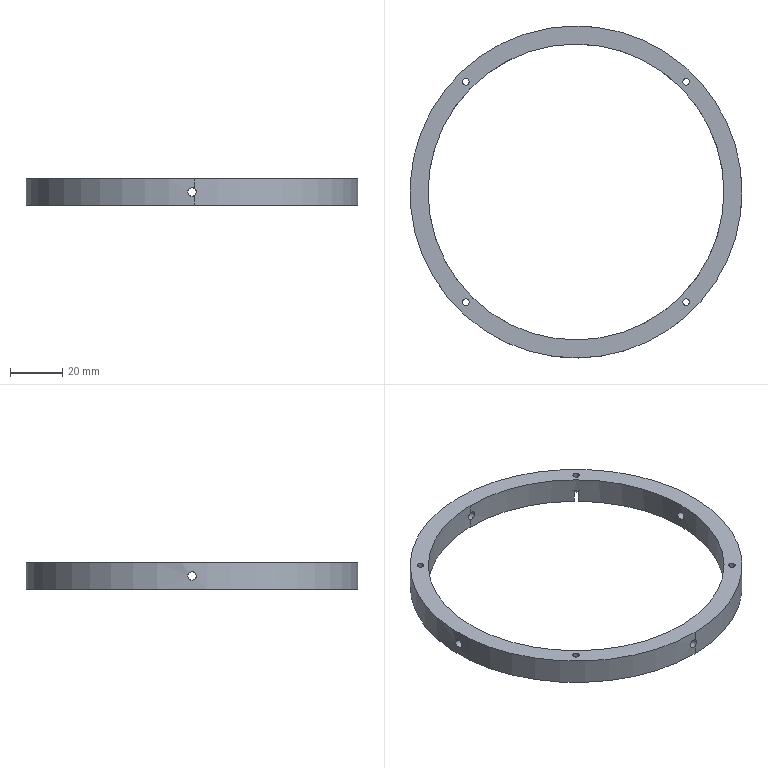CAM job | Mastercam | mm | 6 operations | part box 126.8 x 126.8 x 10
1. Contour (Ramp) | 4 - 4 平铣刀
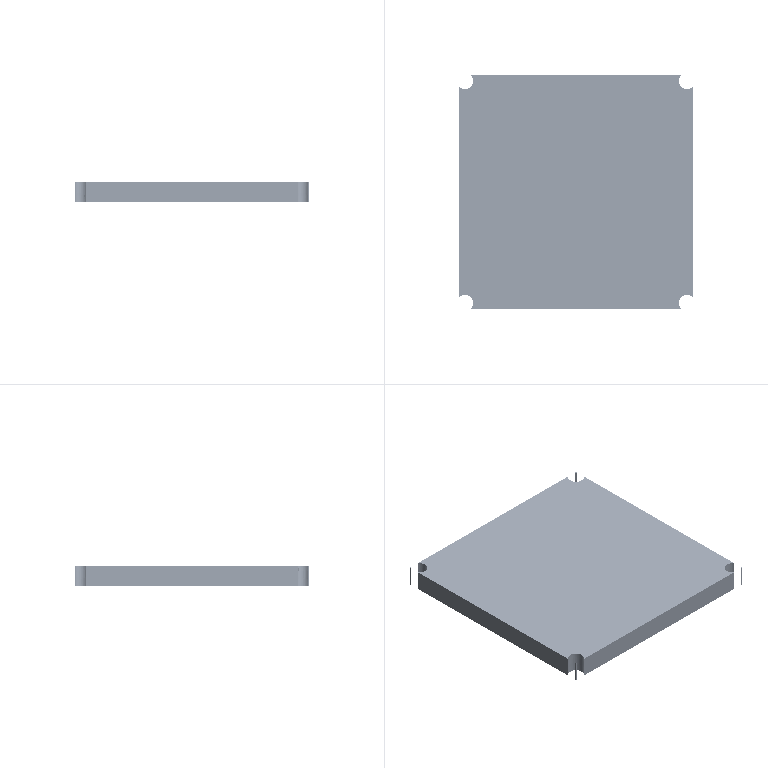2. Contour (2D) | 4 - 4 平铣刀
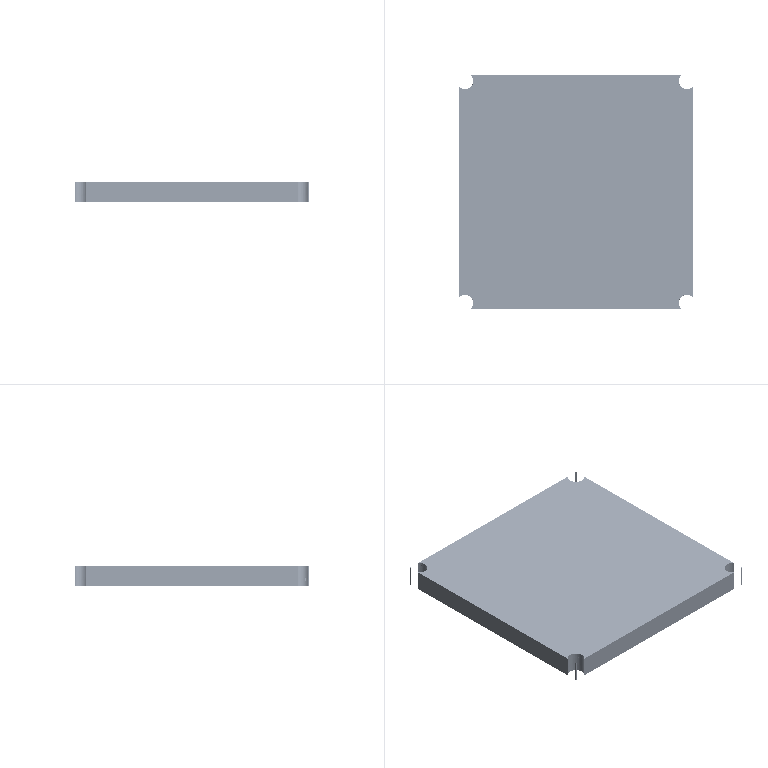3. Contour (2D chamfer) | 7 - 4 倒角刀
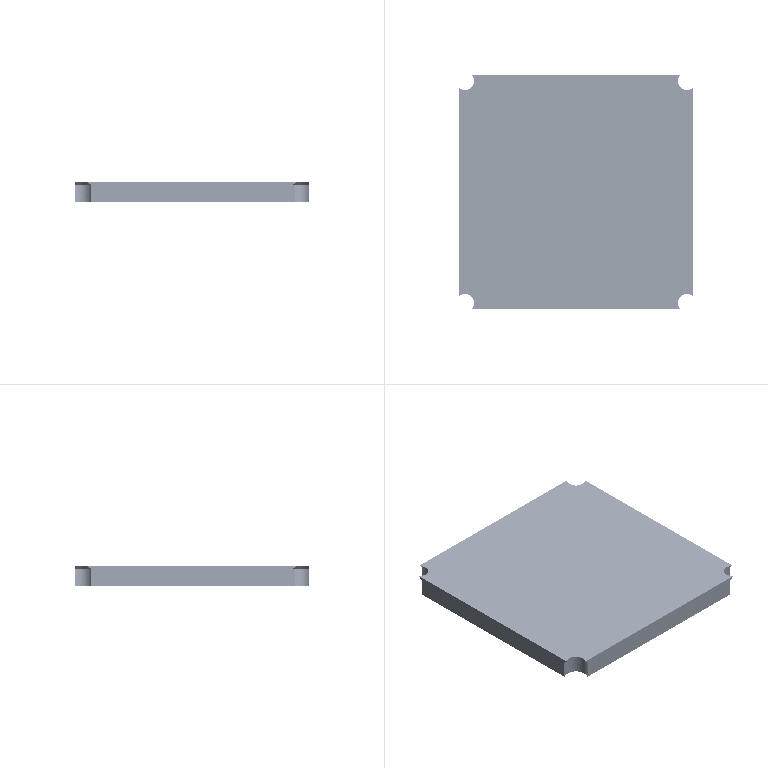4. Drill/Counterbore | 7 - 4 倒角刀
5. Drill/Counterbore | 7 - 4 倒角刀
6. Peck Drill | 1 - 3.3 钻头